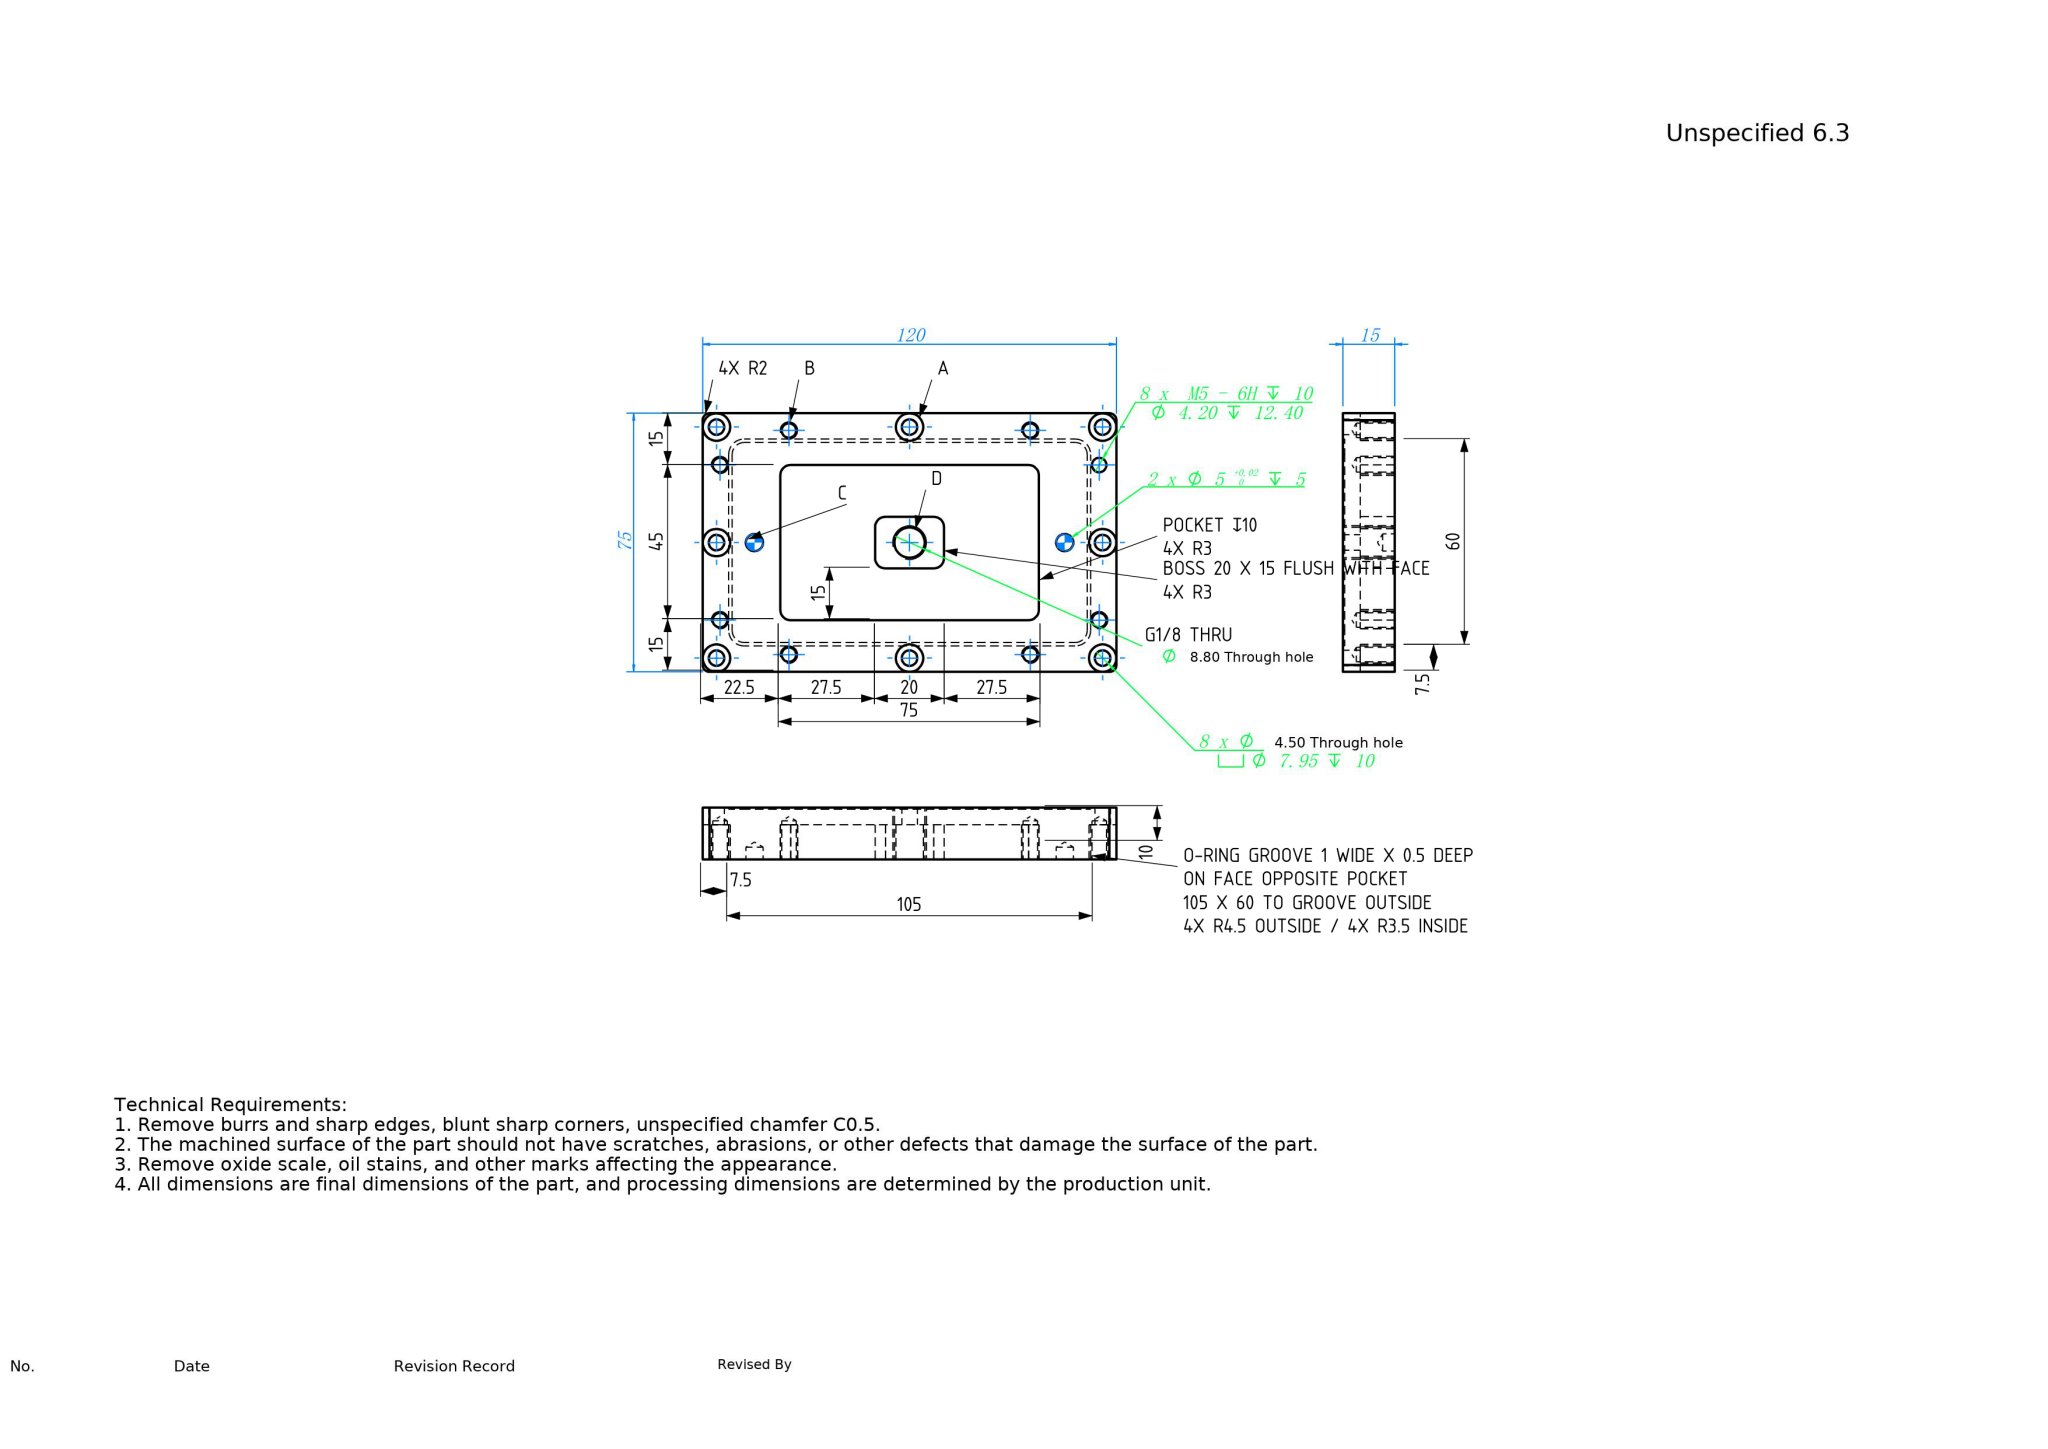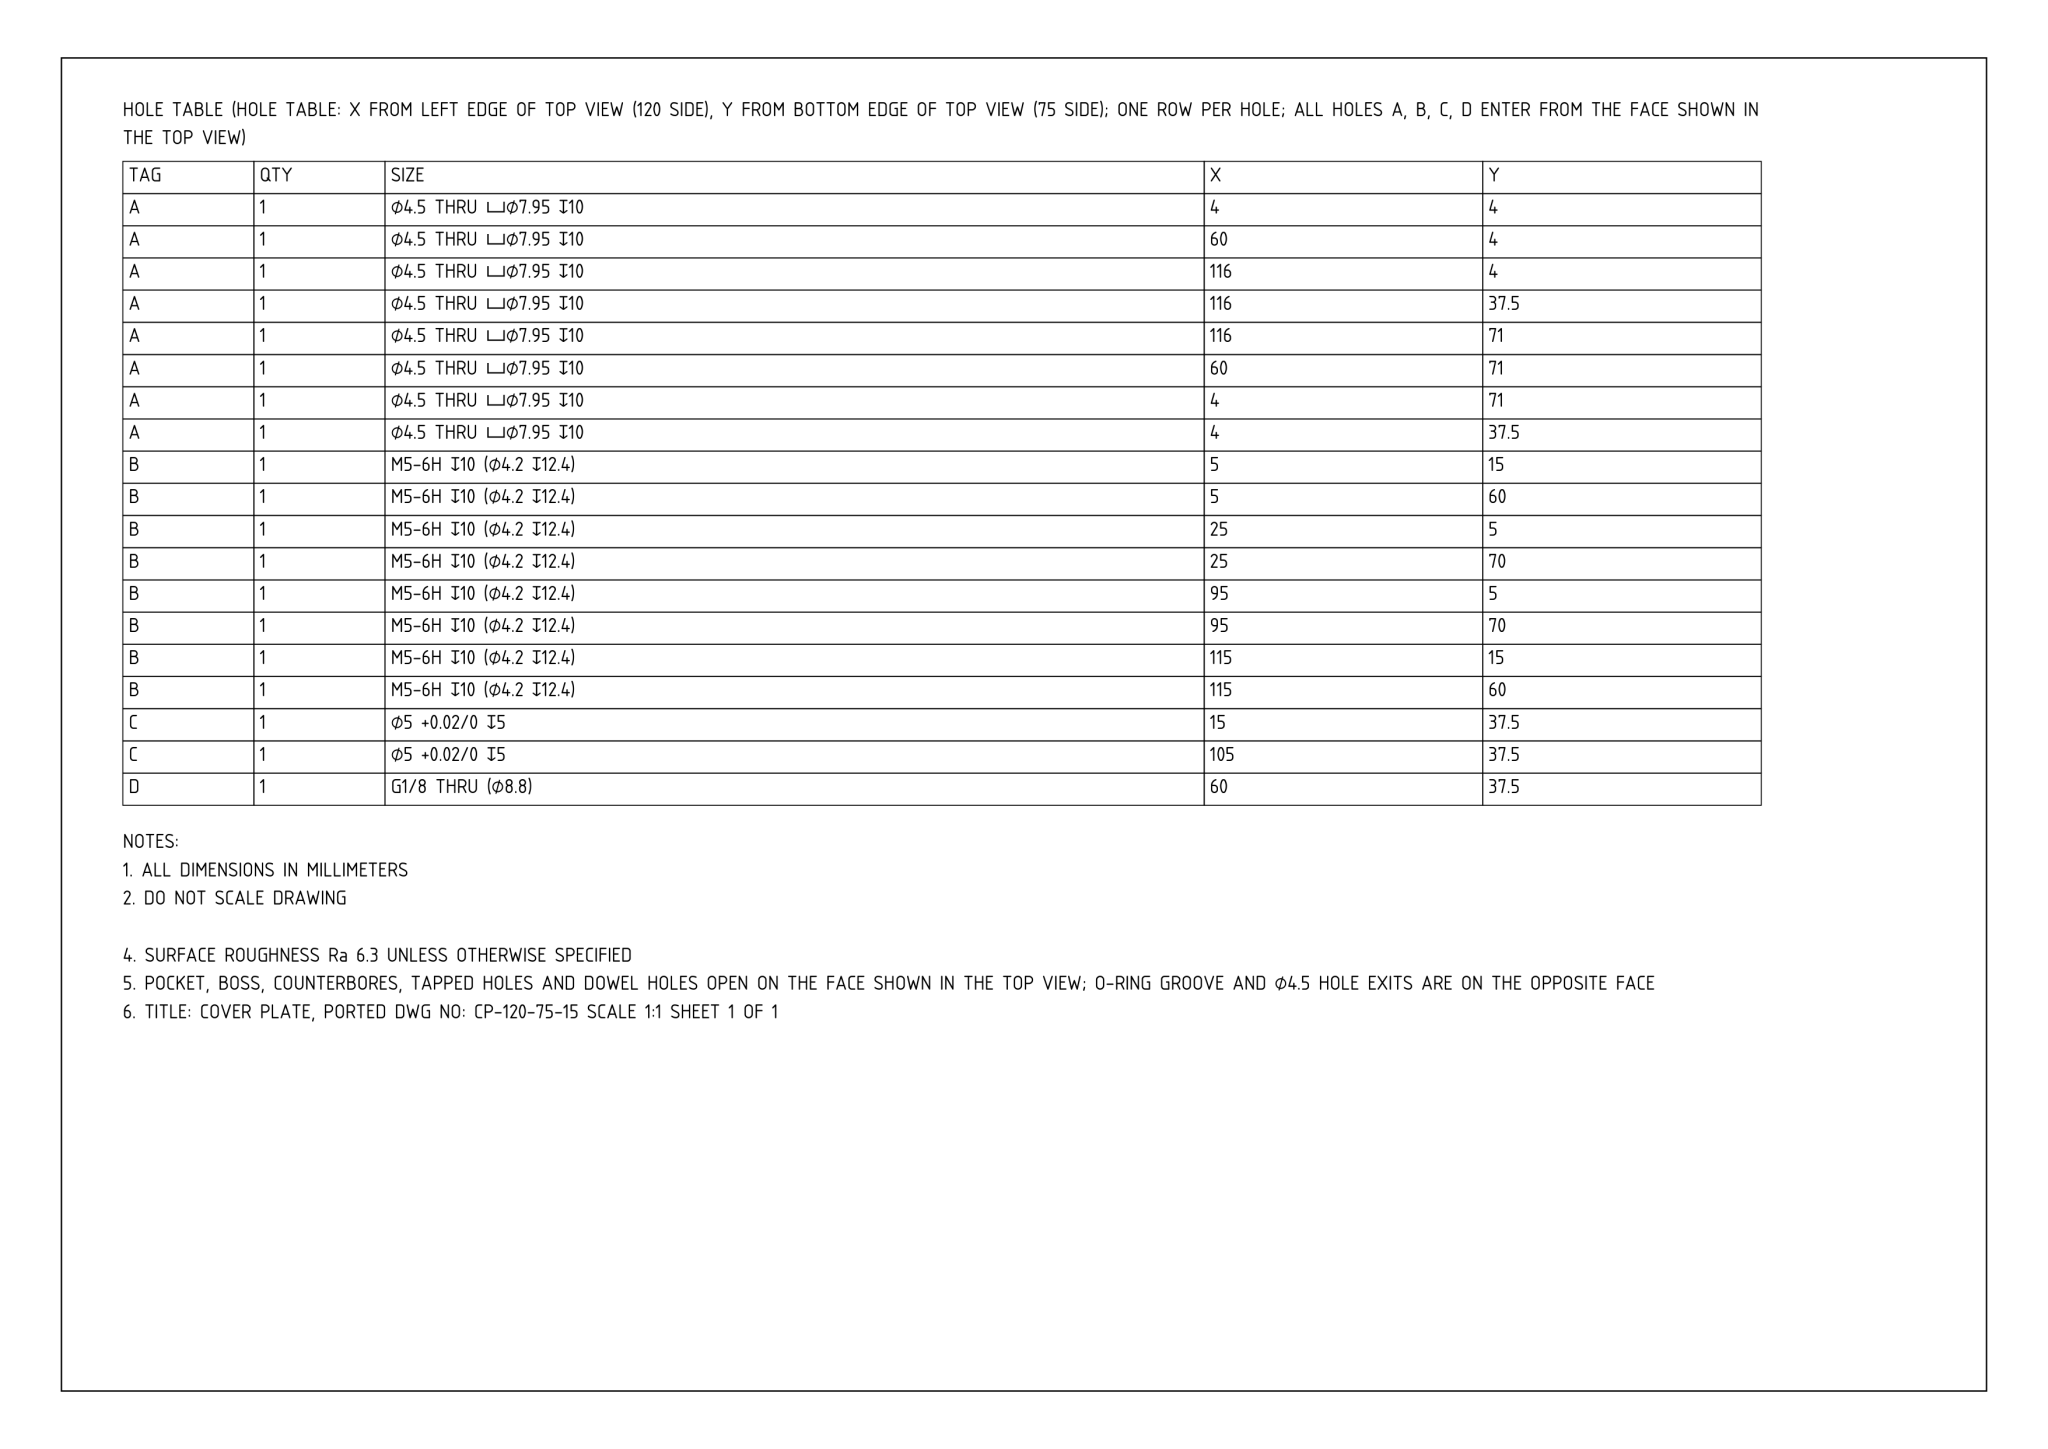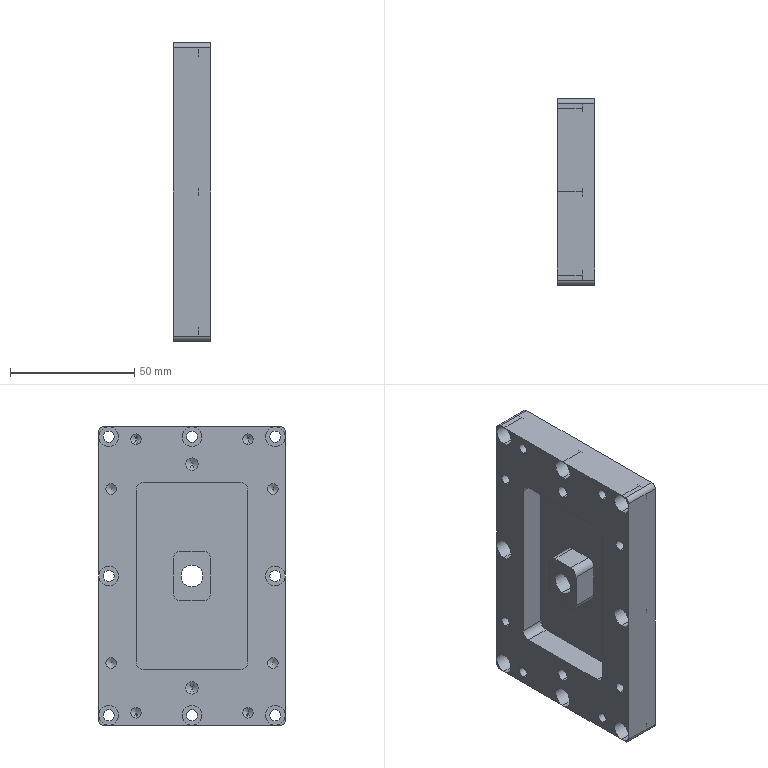Part | NX | mm | 1 solid | 128 faces | box 15 x 75 x 120 mm | volume 97081 mm3 | cylinder 74 | plane 34 | cone 20 | commonest cylinder face diameters 4.2 x16 7.95 x16 4.5 x16 6 x8 5 x4 4 x4 9 x4 7 x4